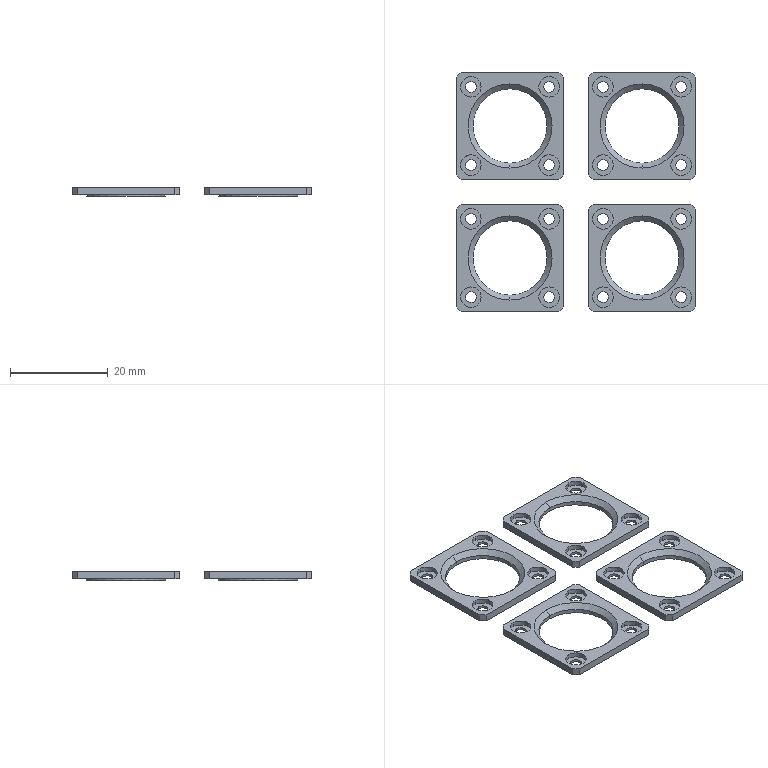CAM job | Mastercam | mm | 12 operations | part box 49 x 49 x 1.8
1. Contour (Ramp) | 1 - 6C
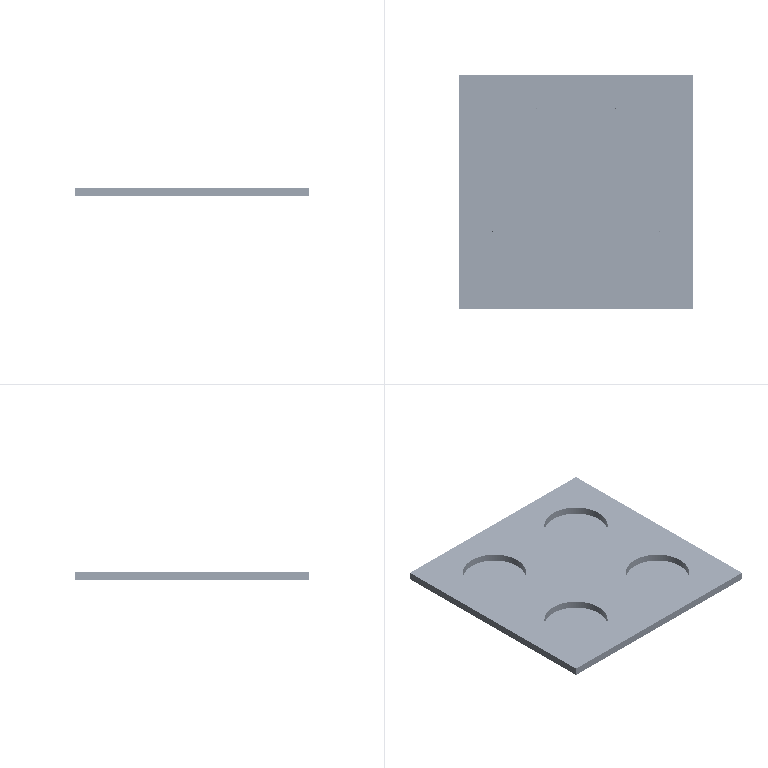2. Contour (2D) | 2 - 6J
3. Contour (Ramp) | 3 - 2C
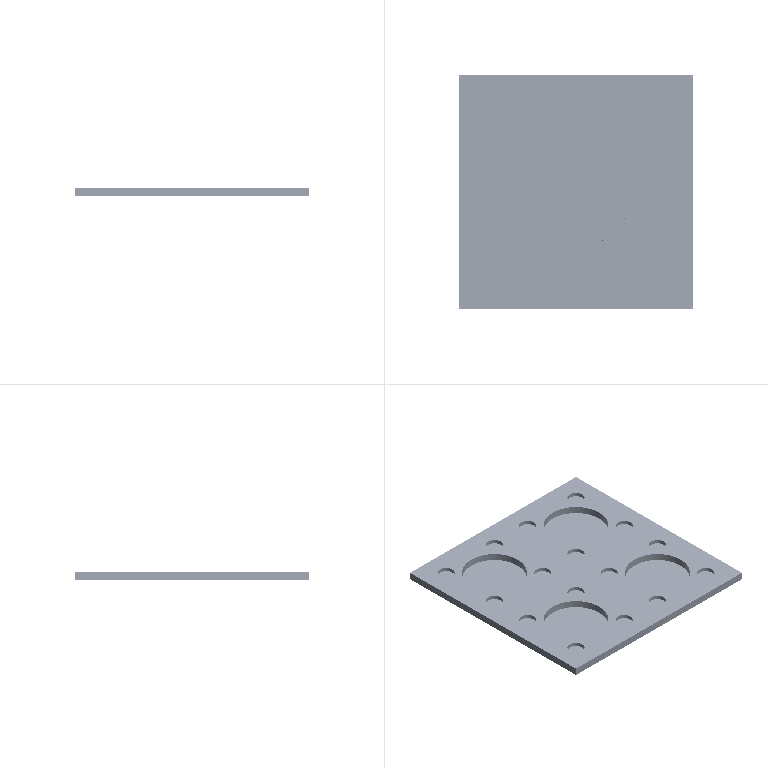4. Contour (Ramp) | 3 - 2C
5. Contour (2D) | 4 - 2J
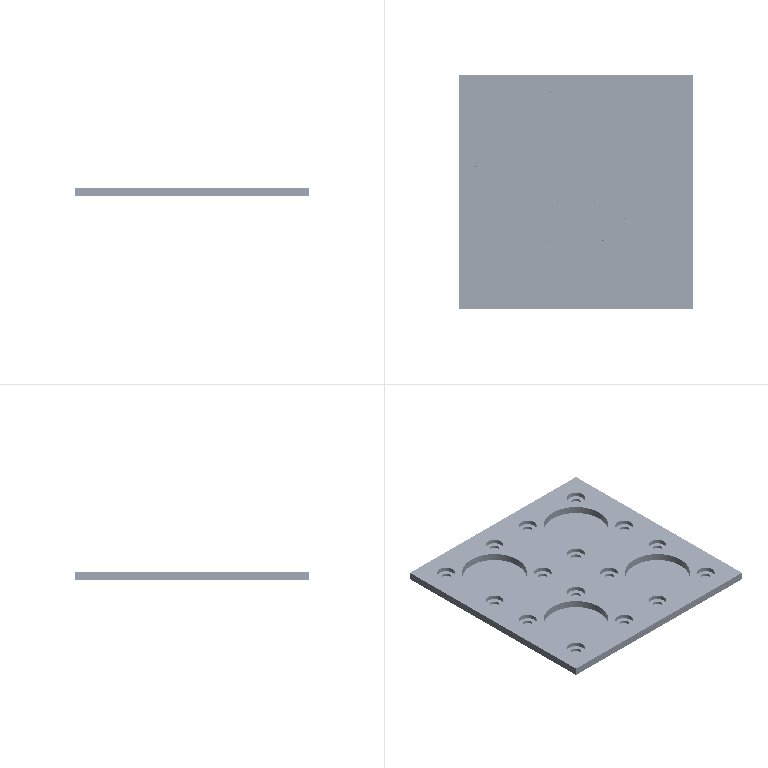6. Contour (2D) | 4 - 2J
7. Contour (2D chamfer) | 5 - 4 倒角刀
8. Contour (2D chamfer) | 5 - 4 倒角刀
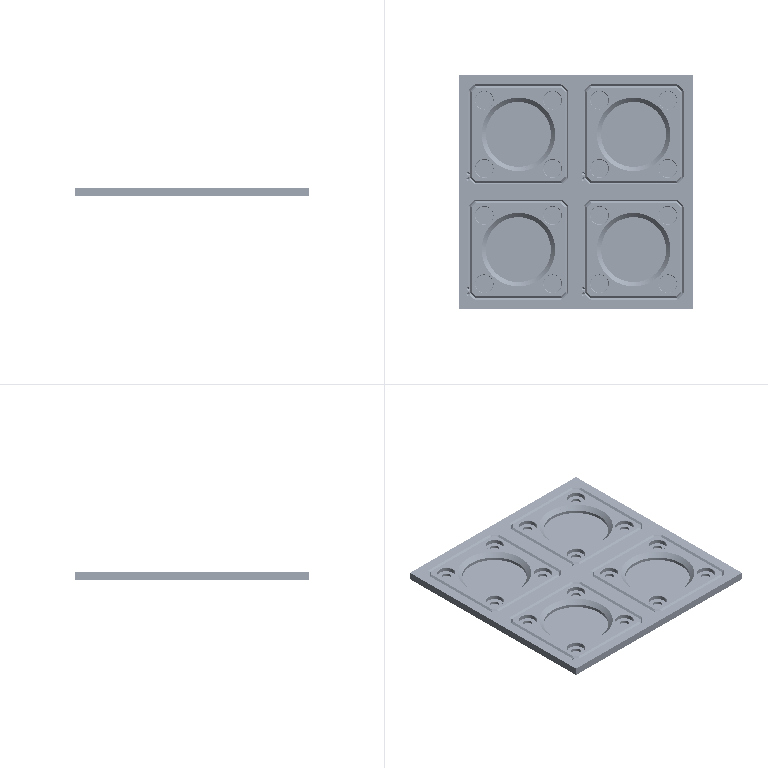9. Contour (Ramp) | 6 - 4C
10. Contour (2D) | 7 - 4J
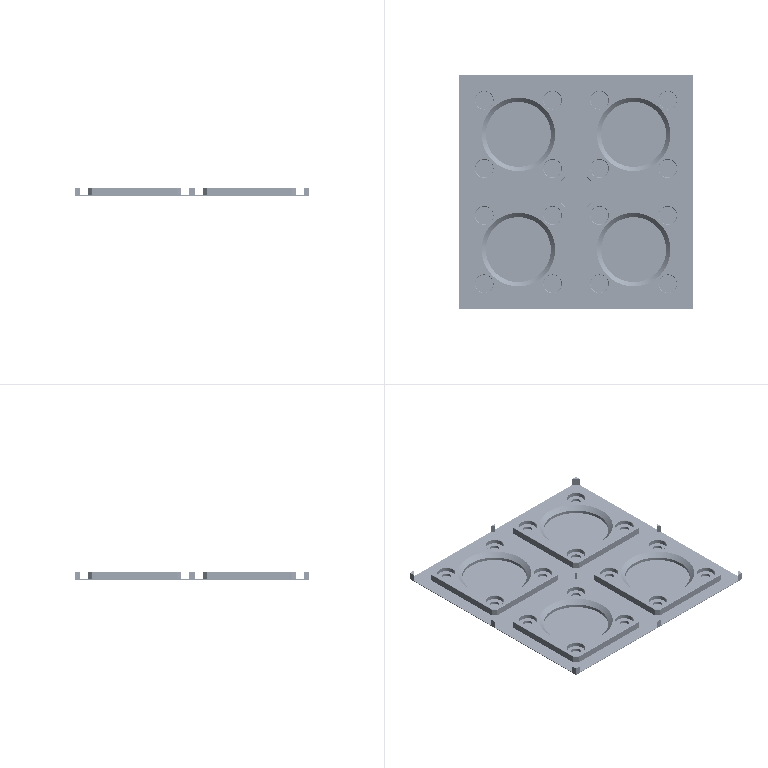11. 2D High Speed (2D Area Mill) | 7 - 4J
12. Model Chamfer | 5 - 4 倒角刀